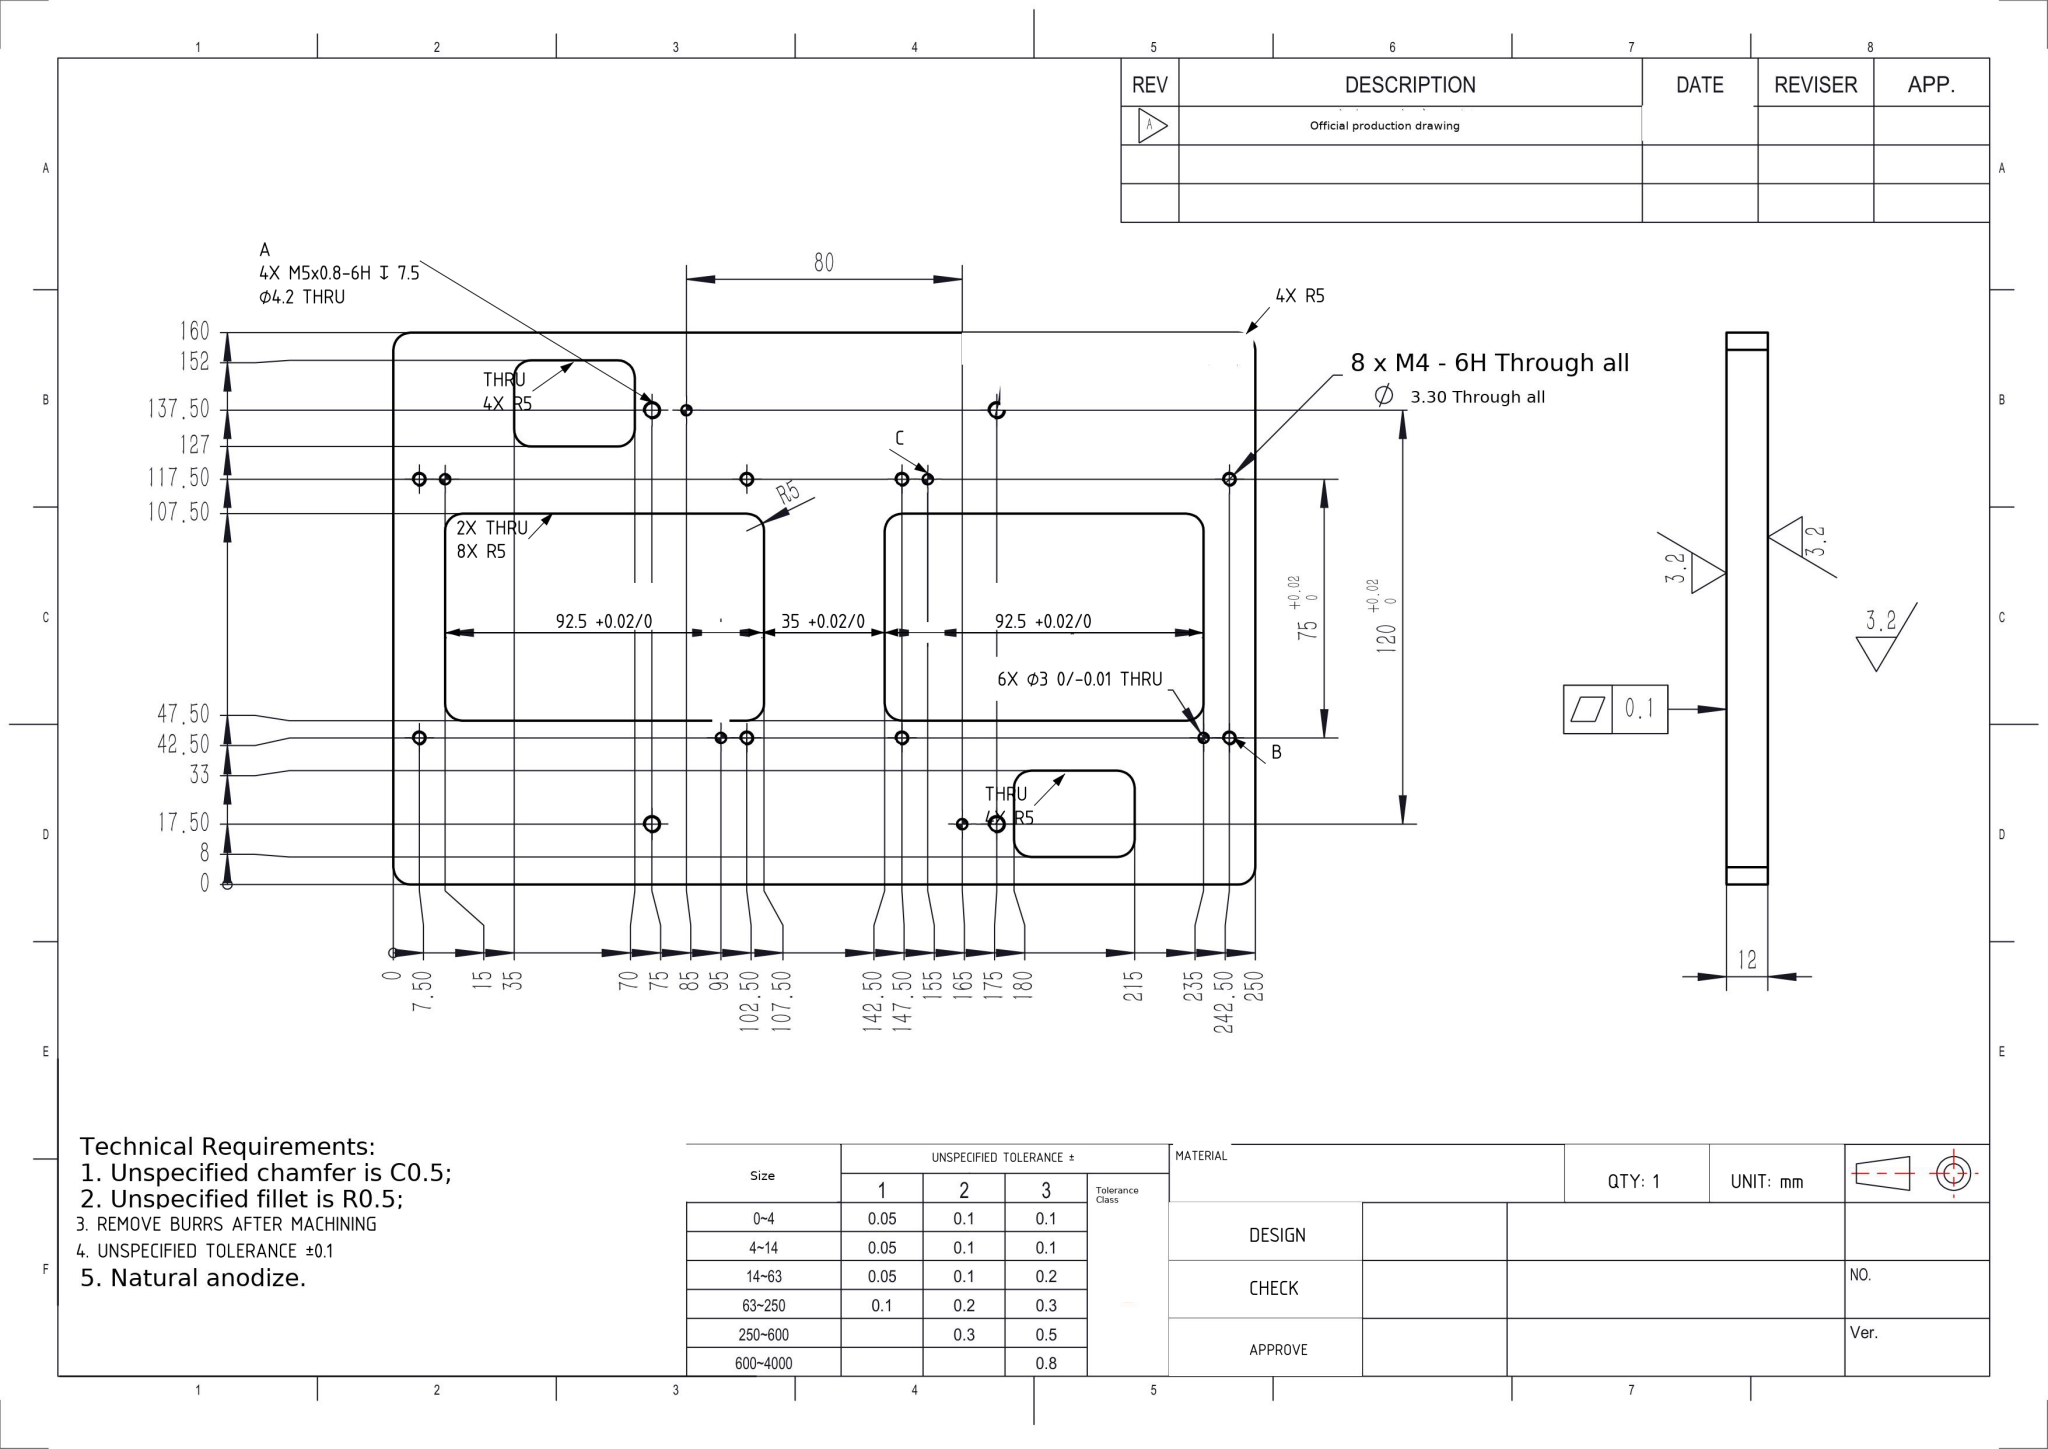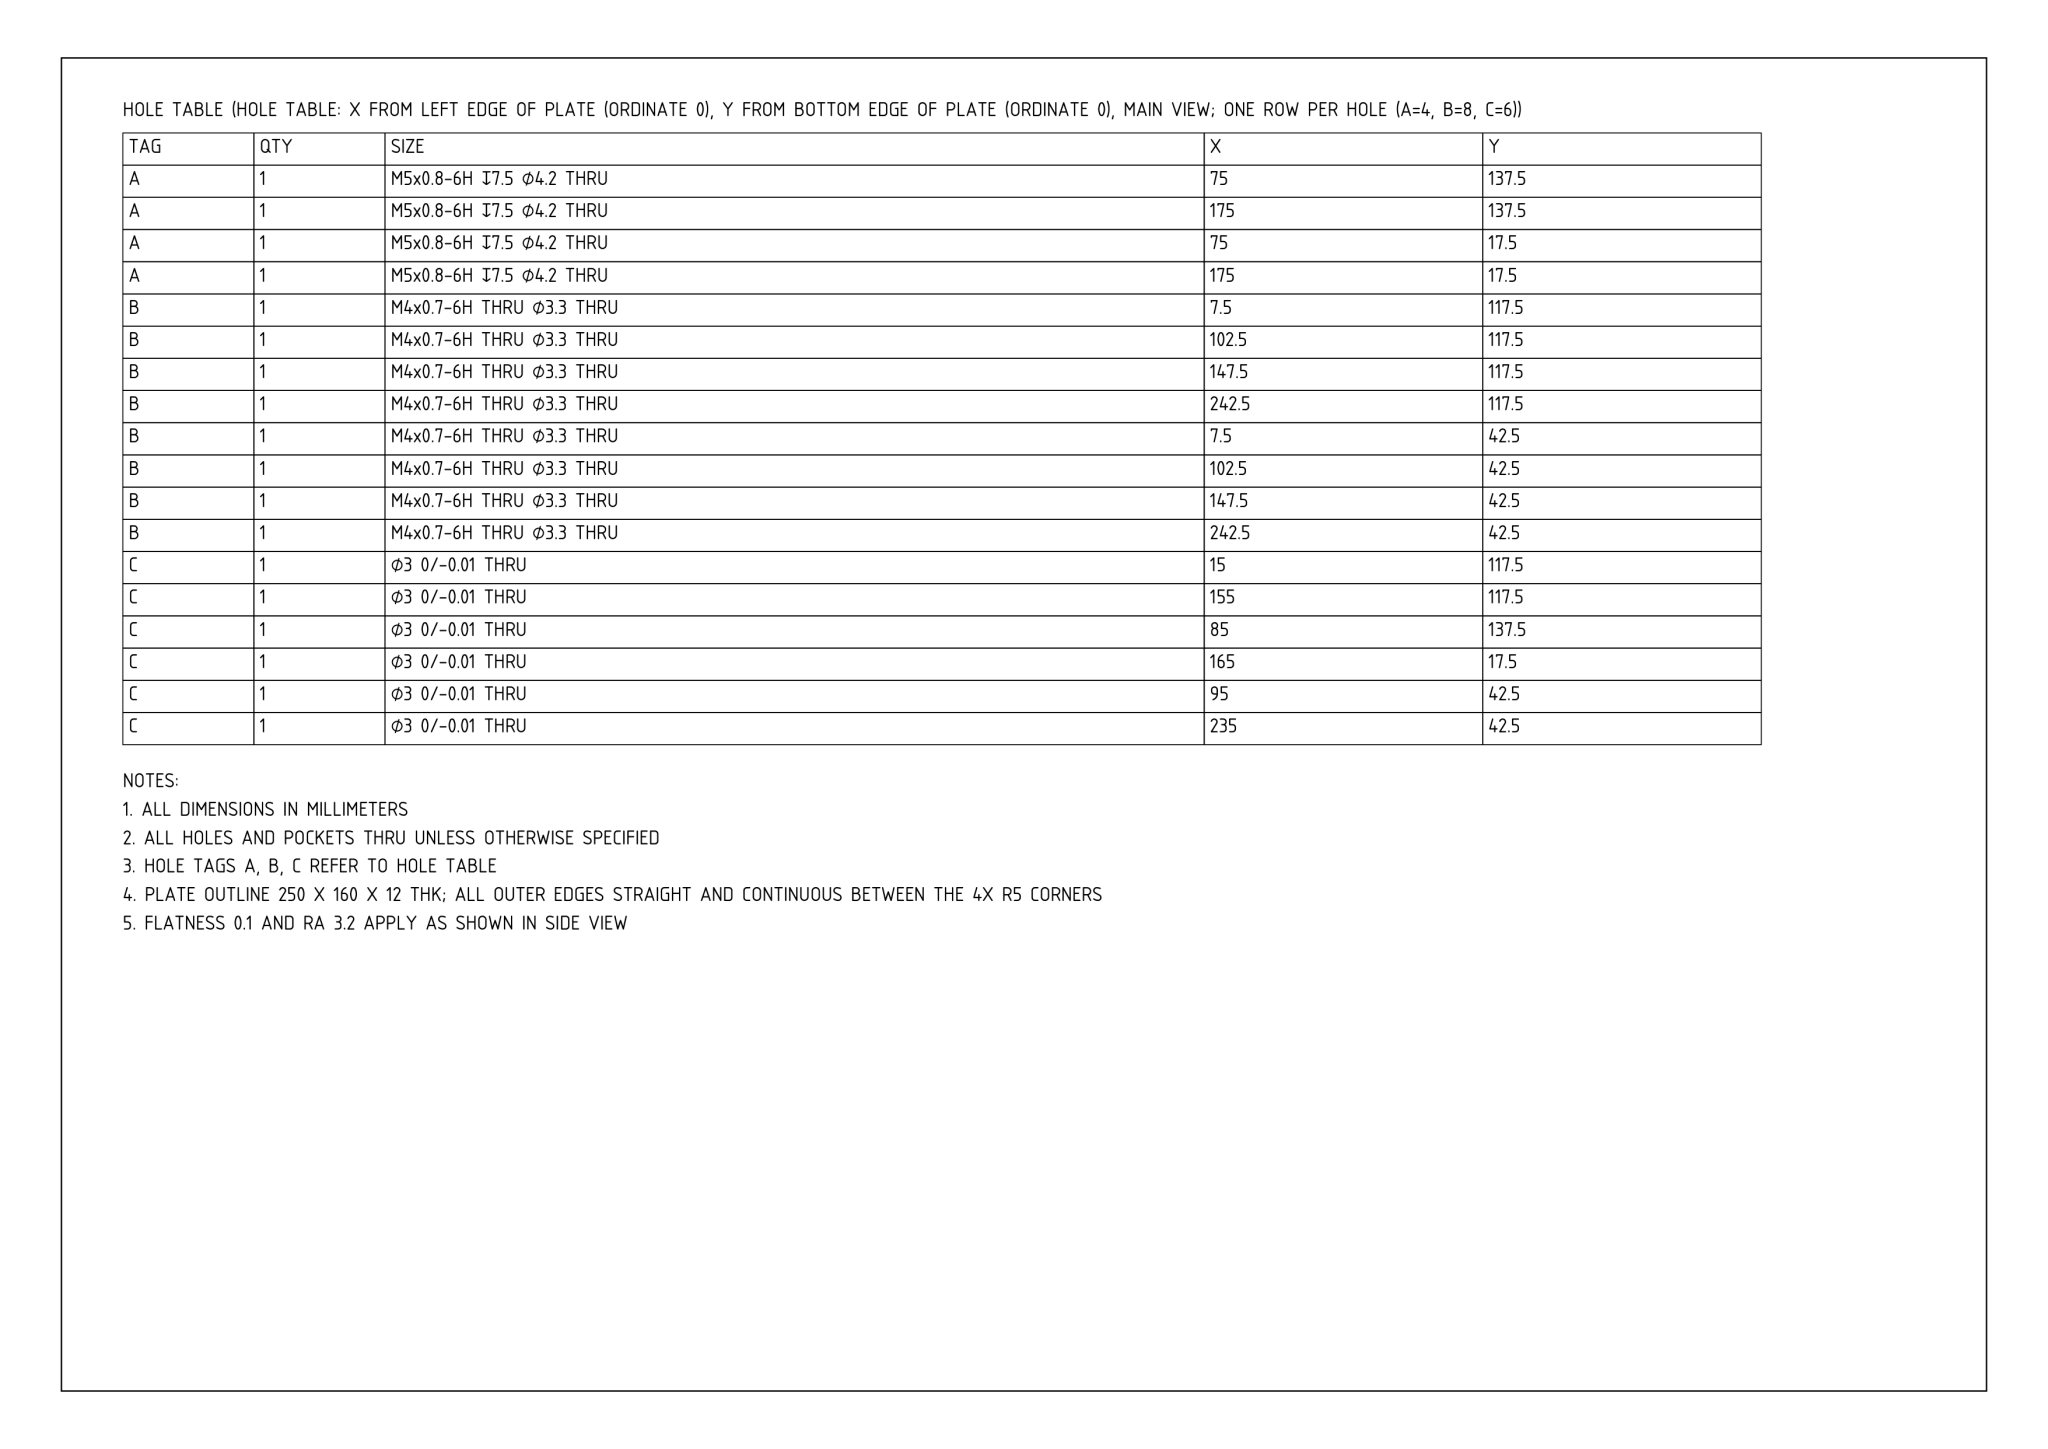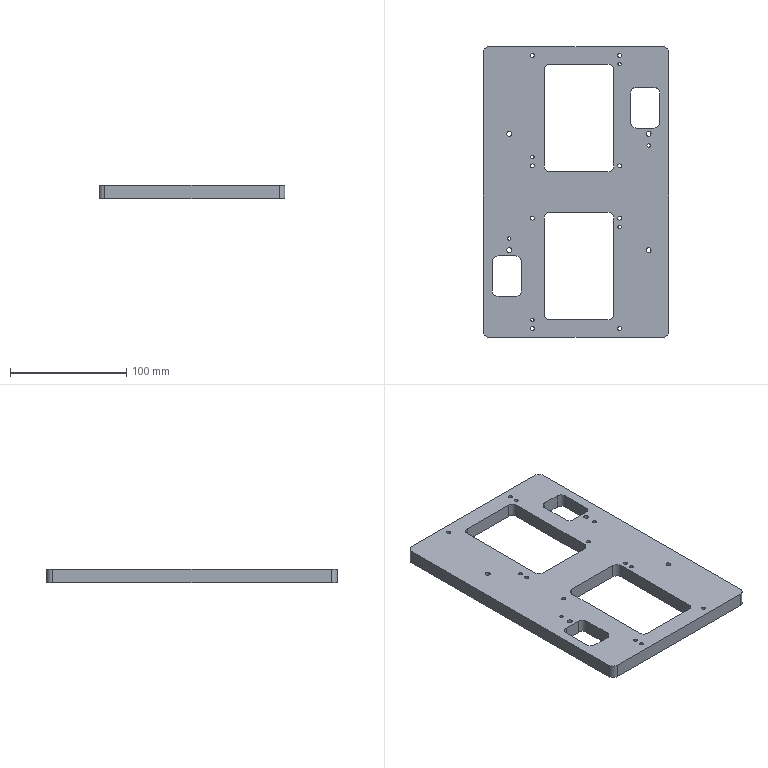Part | NX | mm | 1 solid | 78 faces | box 160 x 250 x 12 mm | volume 324578 mm3 | cylinder 56 | plane 22 | commonest cylinder face diameters 10 x20 3.3 x16 3 x12 4.2 x8